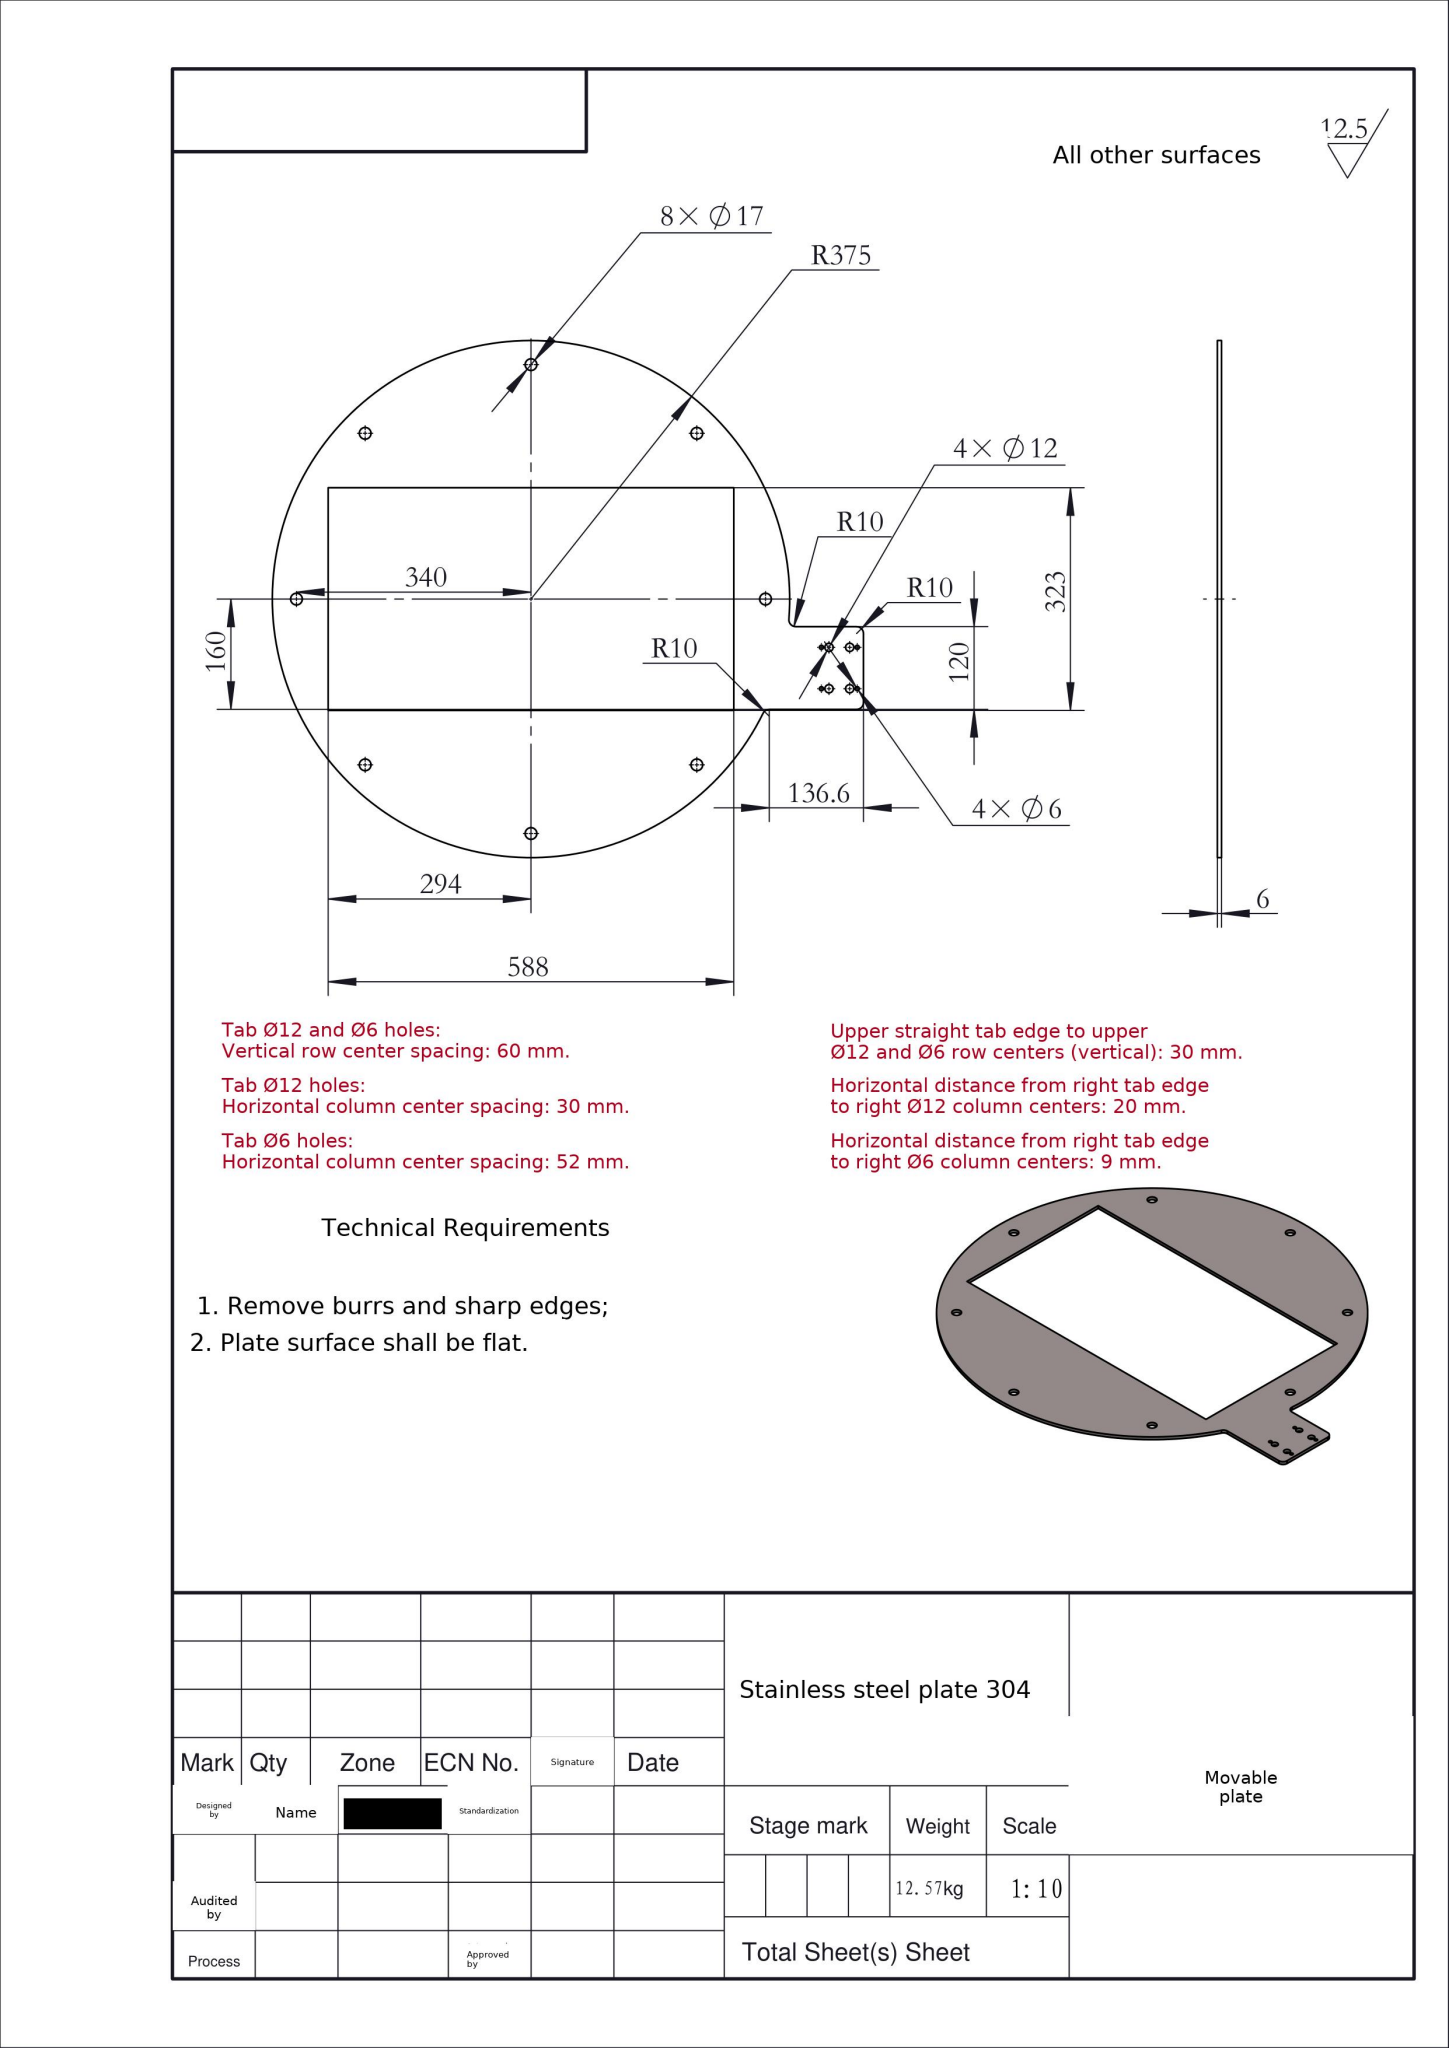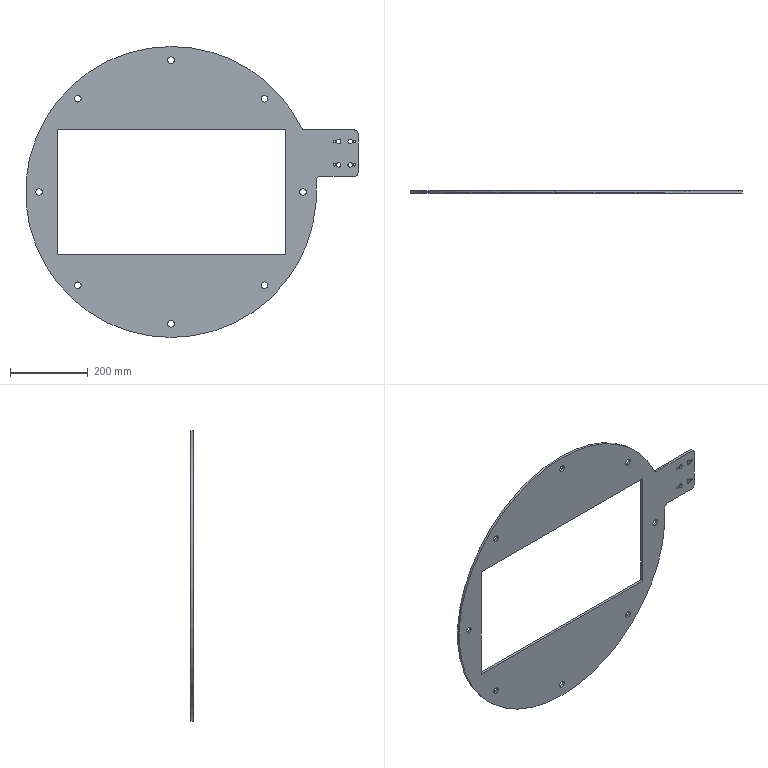Part | SolidWorks | mm | material Stainless steel plate 304 | 1 solid | 48 faces | box 857 x 6 x 750 mm | volume 1584938 mm3 | cylinder 39 | plane 9 | commonest cylinder face diameters 17 x16 12 x8 6 x8 20 x4 750 x3